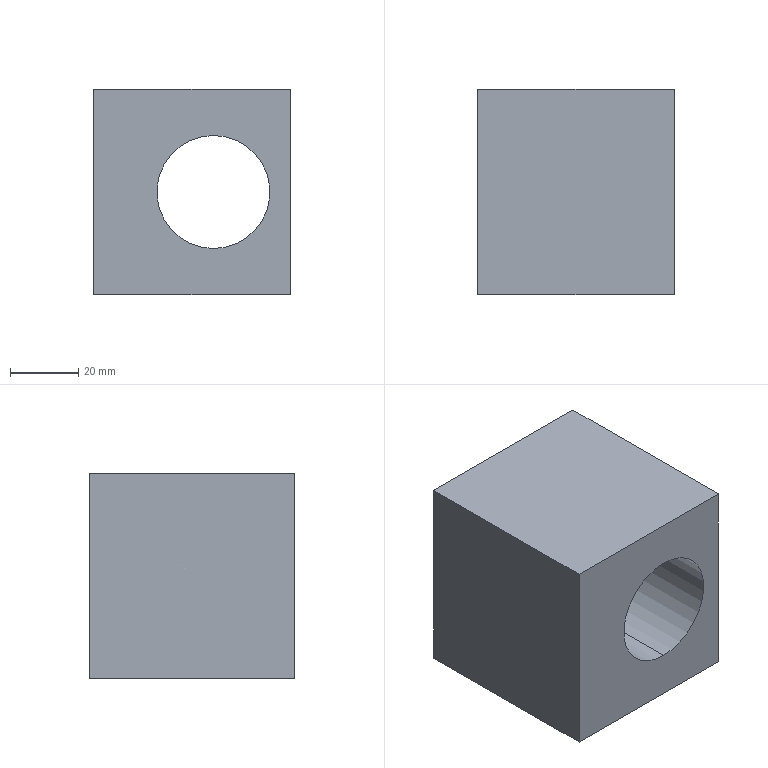Component | SolidWorks | JF21-80.1-1-3(_)-1-SOLID45-1 | 1 solid | 8 faces | box 57.5 x 60 x 60 mm | volume 155682 mm3 | plane 6 | cylinder 2 | commonest cylinder face diameters 33 x2
STEP:
#1=CARTESIAN_POINT('',(18.701,-64.567,-7.146));
#2=VERTEX_POINT('',#1);
#3=CARTESIAN_POINT('',(18.701,-64.567,-5.846));
#4=VERTEX_POINT('',#3);
#5=CARTESIAN_POINT('',(18.701,-64.567,-6.496));
#6=DIRECTION('',(0.,1.,0.));
#7=DIRECTION('',(0.,0.,1.));
#8=AXIS2_PLACEMENT_3D('',#5,#6,#7);
#9=CIRCLE('',#8,0.6496);
#10=EDGE_CURVE('',#2,#4,#9,.T.);
#11=ORIENTED_EDGE('',*,*,#10,.F.);
#12=CARTESIAN_POINT('',(18.701,-62.205,-7.146));
#13=VERTEX_POINT('',#12);
#14=CARTESIAN_POINT('',(18.701,-62.205,-7.146));
#15=DIRECTION('',(0.,1.,0.));
#16=VECTOR('',#15,39.37);
#17=LINE('',#14,#16);
#18=EDGE_CURVE('',#2,#13,#17,.T.);
#19=ORIENTED_EDGE('',*,*,#18,.T.);
#20=CARTESIAN_POINT('',(18.701,-62.205,-5.846));
#21=VERTEX_POINT('',#20);
#22=CARTESIAN_POINT('',(18.701,-62.205,-6.496));
#23=DIRECTION('',(0.,1.,0.));
#24=DIRECTION('',(0.,0.,1.));
#25=AXIS2_PLACEMENT_3D('',#22,#23,#24);
#26=CIRCLE('',#25,0.6496);
#27=EDGE_CURVE('',#13,#21,#26,.T.);
#28=ORIENTED_EDGE('',*,*,#27,.T.);
#29=CARTESIAN_POINT('',(18.701,-62.205,-5.846));
#30=DIRECTION('',(0.,1.,0.));
#31=VECTOR('',#30,39.37);
#32=LINE('',#29,#31);
#33=EDGE_CURVE('',#4,#21,#32,.T.);
#34=ORIENTED_EDGE('',*,*,#33,.F.);
#35=EDGE_LOOP('',(#11,#19,#28,#34));
#36=FACE_OUTER_BOUND('',#35,.T.);
#37=CARTESIAN_POINT('',(18.701,-62.205,-6.496));
#38=DIRECTION('',(0.,1.,0.));
#39=DIRECTION('',(0.,0.,-1.));
#40=AXIS2_PLACEMENT_3D('',#37,#38,#39);
#41=CYLINDRICAL_SURFACE('',#40,0.6496);
#42=ADVANCED_FACE('',(#36),#41,.F.);
#43=CARTESIAN_POINT('',(17.323,-62.205,-7.677));
#44=VERTEX_POINT('',#43);
#45=CARTESIAN_POINT('',(17.323,-62.205,-5.315));
#46=VERTEX_POINT('',#45);
#47=CARTESIAN_POINT('',(17.323,-62.205,-7.677));
#48=DIRECTION('',(0.,0.,1.));
#49=VECTOR('',#48,39.37);
#50=LINE('',#47,#49);
#51=EDGE_CURVE('',#44,#46,#50,.T.);
#52=ORIENTED_EDGE('',*,*,#51,.F.);
#53=CARTESIAN_POINT('',(17.323,-64.567,-7.677));
#54=VERTEX_POINT('',#53);
#55=CARTESIAN_POINT('',(17.323,-64.567,-7.677));
#56=DIRECTION('',(0.,1.,0.));
#57=VECTOR('',#56,39.37);
#58=LINE('',#55,#57);
#59=EDGE_CURVE('',#54,#44,#58,.T.);
#60=ORIENTED_EDGE('',*,*,#59,.F.);
#61=CARTESIAN_POINT('',(17.323,-64.567,-5.315));
#62=VERTEX_POINT('',#61);
#63=CARTESIAN_POINT('',(17.323,-64.567,-7.677));
#64=DIRECTION('',(0.,0.,1.));
#65=VECTOR('',#64,39.37);
#66=LINE('',#63,#65);
#67=EDGE_CURVE('',#54,#62,#66,.T.);
#68=ORIENTED_EDGE('',*,*,#67,.T.);
#69=CARTESIAN_POINT('',(17.323,-64.567,-5.315));
#70=DIRECTION('',(0.,1.,0.));
#71=VECTOR('',#70,39.37);
#72=LINE('',#69,#71);
#73=EDGE_CURVE('',#62,#46,#72,.T.);
#74=ORIENTED_EDGE('',*,*,#73,.T.);
#75=EDGE_LOOP('',(#52,#60,#68,#74));
#76=FACE_OUTER_BOUND('',#75,.T.);
#77=CARTESIAN_POINT('',(17.323,-64.567,-7.677));
#78=DIRECTION('',(-1.,0.,0.));
#79=DIRECTION('',(0.,0.,-1.));
#80=AXIS2_PLACEMENT_3D('',#77,#78,#79);
#81=PLANE('',#80);
#82=ADVANCED_FACE('',(#76),#81,.T.);
#83=CARTESIAN_POINT('',(19.587,-62.205,-7.677));
#84=VERTEX_POINT('',#83);
#85=CARTESIAN_POINT('',(17.323,-62.205,-7.677));
#86=DIRECTION('',(-1.,0.,0.));
#87=VECTOR('',#86,39.37);
#88=LINE('',#85,#87);
#89=EDGE_CURVE('',#84,#44,#88,.T.);
#90=ORIENTED_EDGE('',*,*,#89,.F.);
#91=CARTESIAN_POINT('',(19.587,-64.567,-7.677));
#92=VERTEX_POINT('',#91);
#93=CARTESIAN_POINT('',(19.587,-64.567,-7.677));
#94=DIRECTION('',(0.,1.,0.));
#95=VECTOR('',#94,39.37);
#96=LINE('',#93,#95);
#97=EDGE_CURVE('',#92,#84,#96,.T.);
#98=ORIENTED_EDGE('',*,*,#97,.F.);
#99=CARTESIAN_POINT('',(17.323,-64.567,-7.677));
#100=DIRECTION('',(-1.,0.,0.));
#101=VECTOR('',#100,39.37);
#102=LINE('',#99,#101);
#103=EDGE_CURVE('',#92,#54,#102,.T.);
#104=ORIENTED_EDGE('',*,*,#103,.T.);
#105=ORIENTED_EDGE('',*,*,#59,.T.);
#106=EDGE_LOOP('',(#90,#98,#104,#105));
#107=FACE_OUTER_BOUND('',#106,.T.);
#108=CARTESIAN_POINT('',(17.323,-64.567,-7.677));
#109=DIRECTION('',(0.,0.,-1.));
#110=DIRECTION('',(1.,0.,0.));
#111=AXIS2_PLACEMENT_3D('',#108,#109,#110);
#112=PLANE('',#111);
#113=ADVANCED_FACE('',(#107),#112,.T.);
#114=CARTESIAN_POINT('',(19.587,-62.205,-5.315));
#115=VERTEX_POINT('',#114);
#116=CARTESIAN_POINT('',(19.587,-62.205,-7.677));
#117=DIRECTION('',(0.,0.,-1.));
#118=VECTOR('',#117,39.37);
#119=LINE('',#116,#118);
#120=EDGE_CURVE('',#115,#84,#119,.T.);
#121=ORIENTED_EDGE('',*,*,#120,.F.);
#122=CARTESIAN_POINT('',(19.587,-64.567,-5.315));
#123=VERTEX_POINT('',#122);
#124=CARTESIAN_POINT('',(19.587,-64.567,-5.315));
#125=DIRECTION('',(0.,1.,0.));
#126=VECTOR('',#125,39.37);
#127=LINE('',#124,#126);
#128=EDGE_CURVE('',#123,#115,#127,.T.);
#129=ORIENTED_EDGE('',*,*,#128,.F.);
#130=CARTESIAN_POINT('',(19.587,-64.567,-7.677));
#131=DIRECTION('',(0.,0.,-1.));
#132=VECTOR('',#131,39.37);
#133=LINE('',#130,#132);
#134=EDGE_CURVE('',#123,#92,#133,.T.);
#135=ORIENTED_EDGE('',*,*,#134,.T.);
#136=ORIENTED_EDGE('',*,*,#97,.T.);
#137=EDGE_LOOP('',(#121,#129,#135,#136));
#138=FACE_OUTER_BOUND('',#137,.T.);
#139=CARTESIAN_POINT('',(19.587,-64.567,-7.677));
#140=DIRECTION('',(1.,0.,0.));
#141=DIRECTION('',(0.,0.,1.));
#142=AXIS2_PLACEMENT_3D('',#139,#140,#141);
#143=PLANE('',#142);
#144=ADVANCED_FACE('',(#138),#143,.T.);
#145=CARTESIAN_POINT('',(17.323,-62.205,-5.315));
#146=DIRECTION('',(1.,0.,0.));
#147=VECTOR('',#146,39.37);
#148=LINE('',#145,#147);
#149=EDGE_CURVE('',#46,#115,#148,.T.);
#150=ORIENTED_EDGE('',*,*,#149,.F.);
#151=ORIENTED_EDGE('',*,*,#73,.F.);
#152=CARTESIAN_POINT('',(17.323,-64.567,-5.315));
#153=DIRECTION('',(1.,0.,0.));
#154=VECTOR('',#153,39.37);
#155=LINE('',#152,#154);
#156=EDGE_CURVE('',#62,#123,#155,.T.);
#157=ORIENTED_EDGE('',*,*,#156,.T.);
#158=ORIENTED_EDGE('',*,*,#128,.T.);
#159=EDGE_LOOP('',(#150,#151,#157,#158));
#160=FACE_OUTER_BOUND('',#159,.T.);
#161=CARTESIAN_POINT('',(17.323,-64.567,-5.315));
#162=DIRECTION('',(0.,0.,1.));
#163=DIRECTION('',(-1.,0.,0.));
#164=AXIS2_PLACEMENT_3D('',#161,#162,#163);
#165=PLANE('',#164);
#166=ADVANCED_FACE('',(#160),#165,.T.);
#167=CARTESIAN_POINT('',(18.701,-64.567,-6.496));
#168=DIRECTION('',(0.,1.,0.));
#169=DIRECTION('',(0.,0.,1.));
#170=AXIS2_PLACEMENT_3D('',#167,#168,#169);
#171=CIRCLE('',#170,0.6496);
#172=EDGE_CURVE('',#4,#2,#171,.T.);
#173=ORIENTED_EDGE('',*,*,#172,.T.);
#174=ORIENTED_EDGE('',*,*,#10,.T.);
#175=EDGE_LOOP('',(#173,#174));
#176=FACE_BOUND('',#175,.T.);
#177=ORIENTED_EDGE('',*,*,#67,.F.);
#178=ORIENTED_EDGE('',*,*,#103,.F.);
#179=ORIENTED_EDGE('',*,*,#134,.F.);
#180=ORIENTED_EDGE('',*,*,#156,.F.);
#181=EDGE_LOOP('',(#177,#178,#179,#180));
#182=FACE_OUTER_BOUND('',#181,.T.);
#183=CARTESIAN_POINT('',(17.323,-64.567,-5.315));
#184=DIRECTION('',(0.,1.,0.));
#185=DIRECTION('',(0.,0.,-1.));
#186=AXIS2_PLACEMENT_3D('',#183,#184,#185);
#187=PLANE('',#186);
#188=ADVANCED_FACE('',(#176,#182),#187,.F.);
#189=CARTESIAN_POINT('',(18.701,-62.205,-6.496));
#190=DIRECTION('',(0.,1.,0.));
#191=DIRECTION('',(0.,0.,1.));
#192=AXIS2_PLACEMENT_3D('',#189,#190,#191);
#193=CIRCLE('',#192,0.6496);
#194=EDGE_CURVE('',#21,#13,#193,.T.);
#195=ORIENTED_EDGE('',*,*,#194,.F.);
#196=ORIENTED_EDGE('',*,*,#27,.F.);
#197=EDGE_LOOP('',(#195,#196));
#198=FACE_BOUND('',#197,.T.);
#199=ORIENTED_EDGE('',*,*,#51,.T.);
#200=ORIENTED_EDGE('',*,*,#149,.T.);
#201=ORIENTED_EDGE('',*,*,#120,.T.);
#202=ORIENTED_EDGE('',*,*,#89,.T.);
#203=EDGE_LOOP('',(#199,#200,#201,#202));
#204=FACE_OUTER_BOUND('',#203,.T.);
#205=CARTESIAN_POINT('',(17.323,-62.205,-5.315));
#206=DIRECTION('',(0.,1.,0.));
#207=DIRECTION('',(0.,0.,-1.));
#208=AXIS2_PLACEMENT_3D('',#205,#206,#207);
#209=PLANE('',#208);
#210=ADVANCED_FACE('',(#198,#204),#209,.T.);
#211=ORIENTED_EDGE('',*,*,#18,.F.);
#212=ORIENTED_EDGE('',*,*,#172,.F.);
#213=ORIENTED_EDGE('',*,*,#33,.T.);
#214=ORIENTED_EDGE('',*,*,#194,.T.);
#215=EDGE_LOOP('',(#211,#212,#213,#214));
#216=FACE_OUTER_BOUND('',#215,.T.);
#217=CARTESIAN_POINT('',(18.701,-62.205,-6.496));
#218=DIRECTION('',(0.,1.,0.));
#219=DIRECTION('',(0.,0.,-1.));
#220=AXIS2_PLACEMENT_3D('',#217,#218,#219);
#221=CYLINDRICAL_SURFACE('',#220,0.6496);
#222=ADVANCED_FACE('',(#216),#221,.F.);
#223=CLOSED_SHELL('',(#42,#82,#113,#144,#166,#188,#210,#222));
#224=MANIFOLD_SOLID_BREP('',#223);
#225=CARTESIAN_POINT('',(0.,0.,0.));
#226=DIRECTION('',(0.,0.,1.));
#227=DIRECTION('',(1.,0.,0.));
#228=AXIS2_PLACEMENT_3D('',#225,#226,#227);
#229=(LENGTH_UNIT()NAMED_UNIT(*)SI_UNIT($,.METRE.));
#230=LENGTH_MEASURE_WITH_UNIT(LENGTH_MEASURE(0.0254),#229);
#231=DIMENSIONAL_EXPONENTS(1.,0.,0.,0.,0.,0.,0.);
#232=(CONVERSION_BASED_UNIT('',#230)LENGTH_UNIT()NAMED_UNIT(#231));
#233=UNCERTAINTY_MEASURE_WITH_UNIT(LENGTH_MEASURE(0.00001),#232,'','');
#234=(NAMED_UNIT(*)PLANE_ANGLE_UNIT()SI_UNIT($,.RADIAN.));
#235=(NAMED_UNIT(*)SI_UNIT($,.STERADIAN.)SOLID_ANGLE_UNIT());
#236=(GEOMETRIC_REPRESENTATION_CONTEXT(3)GLOBAL_UNCERTAINTY_ASSIGNED_CONTEXT((#233))GLOBAL_UNIT_ASSIGNED_CONTEXT((#232,#234,#235))REPRESENTATION_CONTEXT('',''));
#237=ADVANCED_BREP_SHAPE_REPRESENTATION('',(#224,#228),#236);
#238=COLOUR_RGB('',0.7922,0.8196,0.9333);
#239=FILL_AREA_STYLE_COLOUR('',#238);
#240=FILL_AREA_STYLE('',(#239));
#241=SURFACE_STYLE_FILL_AREA(#240);
#242=SURFACE_SIDE_STYLE('',(#241));
#243=SURFACE_STYLE_USAGE(.BOTH.,#242);
#244=PRESENTATION_STYLE_ASSIGNMENT((#243));
#245=STYLED_ITEM('',(#244),#224);
#246=(LENGTH_UNIT()NAMED_UNIT(*)SI_UNIT($,.METRE.));
#247=LENGTH_MEASURE_WITH_UNIT(LENGTH_MEASURE(0.0254),#246);
#248=DIMENSIONAL_EXPONENTS(1.,0.,0.,0.,0.,0.,0.);
#249=(CONVERSION_BASED_UNIT('',#247)LENGTH_UNIT()NAMED_UNIT(#248));
#250=UNCERTAINTY_MEASURE_WITH_UNIT(LENGTH_MEASURE(0.00001),#249,'','');
#251=(NAMED_UNIT(*)PLANE_ANGLE_UNIT()SI_UNIT($,.RADIAN.));
#252=(NAMED_UNIT(*)SI_UNIT($,.STERADIAN.)SOLID_ANGLE_UNIT());
#253=(GEOMETRIC_REPRESENTATION_CONTEXT(3)GLOBAL_UNCERTAINTY_ASSIGNED_CONTEXT((#250))GLOBAL_UNIT_ASSIGNED_CONTEXT((#249,#251,#252))REPRESENTATION_CONTEXT('',''));
#254=MECHANICAL_DESIGN_GEOMETRIC_PRESENTATION_REPRESENTATION('',(#245),#253);
#255=PRESENTATION_LAYER_ASSIGNMENT('','',(#245));